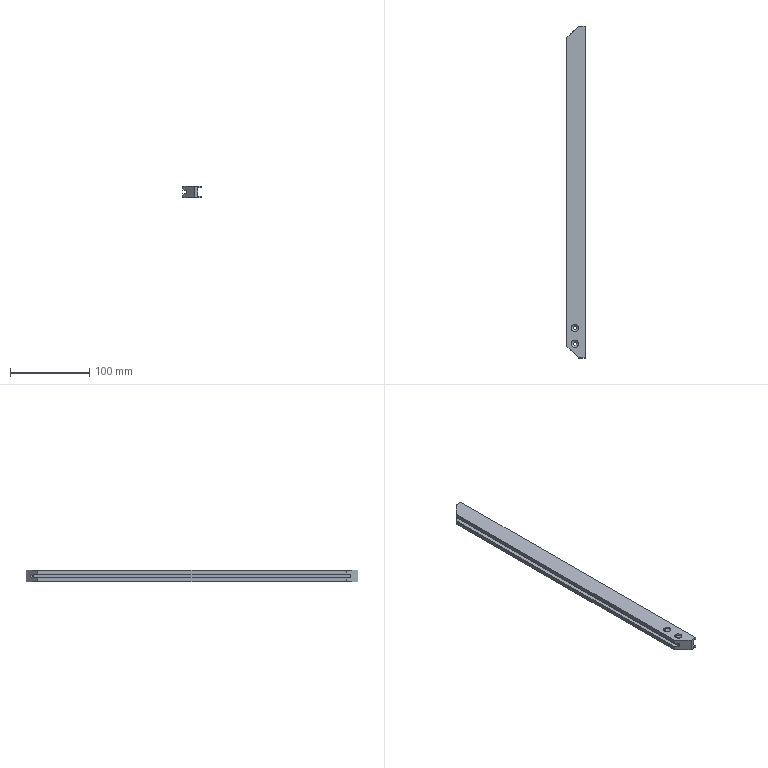Component | SolidWorks | AUTO-SpinDryWashing-01-03000005-1 | 1 solid | 34 faces | box 23 x 420 x 15 mm | volume 113031 mm3 | plane 16 | cylinder 12 | cone 6 | commonest cylinder face diameters 9.4 x4 4.5 x4 3.3 x2 2.5 x2 | material AISI 304
build123d program:
from build123d import *

# Parameters (mm, degrees)
BOSS_EXTRUDE1_DEPTH                                  = 210
CUT_EXTRUDE1_DEPTH                                   = 211.822
COUNTERSUNK_HOLE_FOR_M4_COUNTERSUNK_FLAT_D           = 4.5
COUNTERSUNK_HOLE_FOR_M4_COUNTERSUNK_FLAT_CSINK_D     = 9.4
COUNTERSUNK_HOLE_FOR_M4_COUNTERSUNK_FLAT_CSINK_ANGLE = 90
SKETCH7_W                                            = 15
SKETCH7_H                                            = 420
BOSS_EXTRUDE2_DEPTH                                  = 8
SKETCH8_W                                            = 10.5
SKETCH8_H                                            = 4
CUT_EXTRUDE2_DEPTH                                   = 421.469
M3_TAPPED_HOLE1_D                                    = 2.5
M3_TAPPED_HOLE1_DEPTH                                = 7.5
M3_TAPPED_HOLE1_TIP                                  = 0.7511
BOSS_EXTRUDE3_START                                  = 2
SKETCH12_R                                           = 2.25
BOSS_EXTRUDE3_DEPTH                                  = 2
SKETCH13_R                                           = 4.7
BOSS_EXTRUDE4_DEPTH                                  = 2
M4_TAPPED_HOLE1_D                                    = 3.3


with BuildPart() as part:
    # Sketch1 → Boss-Extrude1 (new, symmetric)
    with BuildSketch(Plane.XY):
        Polygon((0, 15), (0, 0), (11, 0), (11, 15), (8, 15), (8, 10), (3, 10), (3, 15), align=None)
    extrude(amount=BOSS_EXTRUDE1_DEPTH, both=True)

    # Sketch2 → Cut-Extrude1 (cut, through all)
    with BuildSketch(Plane.ZY):
        Polygon((-195, 15), (-210, 15), (-210, 0), align=None)
    cut_extrude1 = extrude(amount=-CUT_EXTRUDE1_DEPTH, mode=Mode.SUBTRACT)

    # Mirror1: Cut-Extrude1 across plane
    add(cut_extrude1.mirror(Plane.XY), mode=Mode.SUBTRACT)

    # Countersunk Hole for M4 Countersunk Flat (through all)
    with Locations(Plane.ZY):
        with Locations((-192, 5), (-172, 5)):
            CounterSinkHole(COUNTERSUNK_HOLE_FOR_M4_COUNTERSUNK_FLAT_D / 2, COUNTERSUNK_HOLE_FOR_M4_COUNTERSUNK_FLAT_CSINK_D / 2, counter_sink_angle=COUNTERSUNK_HOLE_FOR_M4_COUNTERSUNK_FLAT_CSINK_ANGLE)

    # Sketch7 → Boss-Extrude2 (add)
    with BuildSketch(Plane.XZ):
        with Locations((5.5, 0)):
            Rectangle(SKETCH7_W, SKETCH7_H)
    extrude(amount=BOSS_EXTRUDE2_DEPTH)

    # Sketch8 → Cut-Extrude2 (cut, through all)
    with BuildSketch(Plane.XY.offset(210)):
        with Locations((5.5, -6)):
            Rectangle(SKETCH8_W, SKETCH8_H)
    extrude(amount=-CUT_EXTRUDE2_DEPTH, mode=Mode.SUBTRACT)

    # M3 Tapped Hole1
    with Locations(Plane(origin=(0, -4, 0), x_dir=(-1, 0, 0), z_dir=(0, -1, 0))):
        with Locations((-5.5, -185)):
            Hole(M3_TAPPED_HOLE1_D / 2, depth=M3_TAPPED_HOLE1_DEPTH)
            with Locations((0, 0, -(M3_TAPPED_HOLE1_DEPTH + M3_TAPPED_HOLE1_TIP / 2))):  # 118° drill point
                Cone(0, M3_TAPPED_HOLE1_D / 2, M3_TAPPED_HOLE1_TIP, mode=Mode.SUBTRACT)

    # Sketch12 → Boss-Extrude3 (add)
    with BuildSketch(Plane(origin=(11, 0, 0), x_dir=(0, 0, -1), z_dir=(1, 0, 0)).offset(BOSS_EXTRUDE3_START)):
        Polygon((210, 0), (195, 15), (-195, 15), (-210, 0), align=None)
        with Locations(Location((172, 5, 0), (0, 0, 180))):
            Circle(SKETCH12_R, mode=Mode.SUBTRACT)
        with Locations(Location((192, 5, 0), (0, 0, 180))):
            Circle(SKETCH12_R, mode=Mode.SUBTRACT)
    extrude(amount=-BOSS_EXTRUDE3_DEPTH)

    # Sketch13 → Boss-Extrude4 (add)
    with BuildSketch(Plane.ZY):
        Polygon((210, 0), (195, 15), (-195, 15), (-210, 0), align=None)
        with Locations((-192, 5)):
            Circle(SKETCH13_R, mode=Mode.SUBTRACT)
        with Locations((-172, 5)):
            Circle(SKETCH13_R, mode=Mode.SUBTRACT)
    extrude(amount=BOSS_EXTRUDE4_DEPTH)

    # M4 Tapped Hole1 (through all)
    with Locations(Plane(origin=(0, 105, 105), x_dir=(1, 0, 0), z_dir=(0, 0.7071, 0.7071))):
        with Locations((5.5, -138.492)):
            Hole(M4_TAPPED_HOLE1_D / 2)


solid = part.part

# Placed as in the assembly
solid = solid.moved(Location((335, 588, 63), (-90, 0, 90)))
STEP:
#1=COLOUR_RGB('',0.7922,0.8196,0.9333);
#2=FILL_AREA_STYLE_COLOUR('',#1);
#3=FILL_AREA_STYLE('',(#2));
#4=SURFACE_STYLE_FILL_AREA(#3);
#5=SURFACE_SIDE_STYLE('',(#4));
#6=SURFACE_STYLE_USAGE(.BOTH.,#5);
#7=PRESENTATION_STYLE_ASSIGNMENT((#6));
#8=CARTESIAN_POINT('',(13.346,30.611,2.264));
#9=VERTEX_POINT('',#8);
#10=CARTESIAN_POINT('',(13.346,30.795,2.264));
#11=VERTEX_POINT('',#10);
#12=CARTESIAN_POINT('',(13.346,30.611,2.264));
#13=CARTESIAN_POINT('',(13.346,30.611,2.394));
#14=CARTESIAN_POINT('',(13.346,30.795,2.394));
#15=CARTESIAN_POINT('',(13.346,30.795,2.264));
#16=(BOUNDED_CURVE()B_SPLINE_CURVE(3,(#12,#13,#14,#15),.UNSPECIFIED.,.F.,.F.)B_SPLINE_CURVE_WITH_KNOTS((4,4),(3.142,6.283),.UNSPECIFIED.)CURVE()GEOMETRIC_REPRESENTATION_ITEM()RATIONAL_B_SPLINE_CURVE((1.,0.3333,0.3333,1.))REPRESENTATION_ITEM(''));
#17=EDGE_CURVE('',#9,#11,#16,.T.);
#18=ORIENTED_EDGE('',*,*,#17,.F.);
#19=CARTESIAN_POINT('',(12.865,31.093,2.264));
#20=VERTEX_POINT('',#19);
#21=CARTESIAN_POINT('',(12.865,31.093,2.264));
#22=DIRECTION('',(-0.7071,0.7071,-0.));
#23=VECTOR('',#22,39.37);
#24=LINE('',#21,#23);
#25=EDGE_CURVE('',#9,#20,#24,.T.);
#26=ORIENTED_EDGE('',*,*,#25,.T.);
#27=CARTESIAN_POINT('',(12.957,31.185,2.264));
#28=VERTEX_POINT('',#27);
#29=CARTESIAN_POINT('',(12.911,31.139,2.264));
#30=DIRECTION('',(-0.7071,0.7071,-0.));
#31=DIRECTION('',(0.7071,0.7071,0.));
#32=AXIS2_PLACEMENT_3D('',#29,#30,#31);
#33=CIRCLE('',#32,0.06496);
#34=EDGE_CURVE('',#20,#28,#33,.T.);
#35=ORIENTED_EDGE('',*,*,#34,.T.);
#36=CARTESIAN_POINT('',(12.957,31.185,2.264));
#37=DIRECTION('',(-0.7071,0.7071,-0.));
#38=VECTOR('',#37,39.37);
#39=LINE('',#36,#38);
#40=EDGE_CURVE('',#11,#28,#39,.T.);
#41=ORIENTED_EDGE('',*,*,#40,.F.);
#42=EDGE_LOOP('',(#18,#26,#35,#41));
#43=FACE_OUTER_BOUND('',#42,.T.);
#44=CARTESIAN_POINT('',(12.911,31.139,2.264));
#45=DIRECTION('',(-0.7071,0.7071,-0.));
#46=DIRECTION('',(0.7071,0.7071,0.));
#47=AXIS2_PLACEMENT_3D('',#44,#45,#46);
#48=CYLINDRICAL_SURFACE('',#47,0.06496);
#49=ADVANCED_FACE('',(#43),#48,.F.);
#50=CARTESIAN_POINT('',(12.992,16.193,2.559));
#51=VERTEX_POINT('',#50);
#52=CARTESIAN_POINT('',(12.992,16.563,2.559));
#53=VERTEX_POINT('',#52);
#54=CARTESIAN_POINT('',(12.992,16.378,2.559));
#55=DIRECTION('',(-0.,-0.,1.));
#56=DIRECTION('',(0.,1.,0.));
#57=AXIS2_PLACEMENT_3D('',#54,#55,#56);
#58=CIRCLE('',#57,0.185);
#59=EDGE_CURVE('',#51,#53,#58,.T.);
#60=ORIENTED_EDGE('',*,*,#59,.T.);
#61=CARTESIAN_POINT('',(12.992,16.563,2.48));
#62=VERTEX_POINT('',#61);
#63=CARTESIAN_POINT('',(12.992,16.563,2.559));
#64=DIRECTION('',(0.,0.,-1.));
#65=VECTOR('',#64,39.37);
#66=LINE('',#63,#65);
#67=EDGE_CURVE('',#53,#62,#66,.T.);
#68=ORIENTED_EDGE('',*,*,#67,.T.);
#69=CARTESIAN_POINT('',(12.992,16.193,2.48));
#70=VERTEX_POINT('',#69);
#71=CARTESIAN_POINT('',(12.992,16.378,2.48));
#72=DIRECTION('',(-0.,-0.,1.));
#73=DIRECTION('',(0.,1.,0.));
#74=AXIS2_PLACEMENT_3D('',#71,#72,#73);
#75=CIRCLE('',#74,0.185);
#76=EDGE_CURVE('',#70,#62,#75,.T.);
#77=ORIENTED_EDGE('',*,*,#76,.F.);
#78=CARTESIAN_POINT('',(12.992,16.193,2.559));
#79=DIRECTION('',(0.,0.,-1.));
#80=VECTOR('',#79,39.37);
#81=LINE('',#78,#80);
#82=EDGE_CURVE('',#51,#70,#81,.T.);
#83=ORIENTED_EDGE('',*,*,#82,.F.);
#84=EDGE_LOOP('',(#60,#68,#77,#83));
#85=FACE_OUTER_BOUND('',#84,.T.);
#86=CARTESIAN_POINT('',(12.992,16.378,2.559));
#87=DIRECTION('',(0.,0.,-1.));
#88=DIRECTION('',(0.,-1.,0.));
#89=AXIS2_PLACEMENT_3D('',#86,#87,#88);
#90=CYLINDRICAL_SURFACE('',#89,0.185);
#91=ADVANCED_FACE('',(#85),#90,.F.);
#92=CARTESIAN_POINT('',(12.992,15.406,2.559));
#93=VERTEX_POINT('',#92);
#94=CARTESIAN_POINT('',(12.992,15.776,2.559));
#95=VERTEX_POINT('',#94);
#96=CARTESIAN_POINT('',(12.992,15.591,2.559));
#97=DIRECTION('',(-0.,-0.,1.));
#98=DIRECTION('',(0.,1.,0.));
#99=AXIS2_PLACEMENT_3D('',#96,#97,#98);
#100=CIRCLE('',#99,0.185);
#101=EDGE_CURVE('',#93,#95,#100,.T.);
#102=ORIENTED_EDGE('',*,*,#101,.T.);
#103=CARTESIAN_POINT('',(12.992,15.776,2.48));
#104=VERTEX_POINT('',#103);
#105=CARTESIAN_POINT('',(12.992,15.776,2.559));
#106=DIRECTION('',(0.,0.,-1.));
#107=VECTOR('',#106,39.37);
#108=LINE('',#105,#107);
#109=EDGE_CURVE('',#95,#104,#108,.T.);
#110=ORIENTED_EDGE('',*,*,#109,.T.);
#111=CARTESIAN_POINT('',(12.992,15.406,2.48));
#112=VERTEX_POINT('',#111);
#113=CARTESIAN_POINT('',(12.992,15.591,2.48));
#114=DIRECTION('',(-0.,-0.,1.));
#115=DIRECTION('',(0.,1.,0.));
#116=AXIS2_PLACEMENT_3D('',#113,#114,#115);
#117=CIRCLE('',#116,0.185);
#118=EDGE_CURVE('',#112,#104,#117,.T.);
#119=ORIENTED_EDGE('',*,*,#118,.F.);
#120=CARTESIAN_POINT('',(12.992,15.406,2.559));
#121=DIRECTION('',(0.,0.,-1.));
#122=VECTOR('',#121,39.37);
#123=LINE('',#120,#122);
#124=EDGE_CURVE('',#93,#112,#123,.T.);
#125=ORIENTED_EDGE('',*,*,#124,.F.);
#126=EDGE_LOOP('',(#102,#110,#119,#125));
#127=FACE_OUTER_BOUND('',#126,.T.);
#128=CARTESIAN_POINT('',(12.992,15.591,2.559));
#129=DIRECTION('',(0.,0.,-1.));
#130=DIRECTION('',(0.,-1.,0.));
#131=AXIS2_PLACEMENT_3D('',#128,#129,#130);
#132=CYLINDRICAL_SURFACE('',#131,0.185);
#133=ADVANCED_FACE('',(#127),#132,.F.);
#134=CARTESIAN_POINT('',(13.051,30.482,2.264));
#135=VERTEX_POINT('',#134);
#136=CARTESIAN_POINT('',(13.051,30.384,2.264));
#137=VERTEX_POINT('',#136);
#138=CARTESIAN_POINT('',(13.051,30.433,2.264));
#139=DIRECTION('',(1.,0.,0.));
#140=DIRECTION('',(0.,-1.,0.));
#141=AXIS2_PLACEMENT_3D('',#138,#139,#140);
#142=CIRCLE('',#141,0.04921);
#143=EDGE_CURVE('',#135,#137,#142,.T.);
#144=ORIENTED_EDGE('',*,*,#143,.F.);
#145=CARTESIAN_POINT('',(13.346,30.482,2.264));
#146=VERTEX_POINT('',#145);
#147=CARTESIAN_POINT('',(13.346,30.482,2.264));
#148=DIRECTION('',(1.,0.,0.));
#149=VECTOR('',#148,39.37);
#150=LINE('',#147,#149);
#151=EDGE_CURVE('',#135,#146,#150,.T.);
#152=ORIENTED_EDGE('',*,*,#151,.T.);
#153=CARTESIAN_POINT('',(13.346,30.384,2.264));
#154=VERTEX_POINT('',#153);
#155=CARTESIAN_POINT('',(13.346,30.433,2.264));
#156=DIRECTION('',(1.,0.,0.));
#157=DIRECTION('',(0.,-1.,0.));
#158=AXIS2_PLACEMENT_3D('',#155,#156,#157);
#159=CIRCLE('',#158,0.04921);
#160=EDGE_CURVE('',#146,#154,#159,.T.);
#161=ORIENTED_EDGE('',*,*,#160,.T.);
#162=CARTESIAN_POINT('',(13.346,30.384,2.264));
#163=DIRECTION('',(1.,0.,0.));
#164=VECTOR('',#163,39.37);
#165=LINE('',#162,#164);
#166=EDGE_CURVE('',#137,#154,#165,.T.);
#167=ORIENTED_EDGE('',*,*,#166,.F.);
#168=EDGE_LOOP('',(#144,#152,#161,#167));
#169=FACE_OUTER_BOUND('',#168,.T.);
#170=CARTESIAN_POINT('',(13.346,30.433,2.264));
#171=DIRECTION('',(1.,0.,0.));
#172=DIRECTION('',(0.,-1.,0.));
#173=AXIS2_PLACEMENT_3D('',#170,#171,#172);
#174=CYLINDRICAL_SURFACE('',#173,0.04921);
#175=ADVANCED_FACE('',(#169),#174,.F.);
#176=CARTESIAN_POINT('',(13.022,30.433,2.264));
#177=VERTEX_POINT('',#176);
#178=CARTESIAN_POINT('',(13.051,30.384,2.264));
#179=DIRECTION('',(0.515,-0.8572,0.));
#180=VECTOR('',#179,39.37);
#181=LINE('',#178,#180);
#182=EDGE_CURVE('',#177,#137,#181,.T.);
#183=ORIENTED_EDGE('',*,*,#182,.F.);
#184=CARTESIAN_POINT('',(13.051,30.482,2.264));
#185=DIRECTION('',(0.515,0.8572,-0.));
#186=VECTOR('',#185,39.37);
#187=LINE('',#184,#186);
#188=EDGE_CURVE('',#177,#135,#187,.T.);
#189=ORIENTED_EDGE('',*,*,#188,.T.);
#190=ORIENTED_EDGE('',*,*,#143,.T.);
#191=EDGE_LOOP('',(#183,#189,#190));
#192=FACE_OUTER_BOUND('',#191,.T.);
#193=CARTESIAN_POINT('',(13.051,30.433,2.264));
#194=DIRECTION('',(1.,0.,0.));
#195=DIRECTION('',(0.,-1.,0.));
#196=AXIS2_PLACEMENT_3D('',#193,#194,#195);
#197=CONICAL_SURFACE('',#196,0.04921,1.03);
#198=ADVANCED_FACE('',(#192),#197,.F.);
#199=CARTESIAN_POINT('',(12.992,15.502,2.384));
#200=VERTEX_POINT('',#199);
#201=CARTESIAN_POINT('',(12.992,15.679,2.384));
#202=VERTEX_POINT('',#201);
#203=CARTESIAN_POINT('',(12.992,15.591,2.384));
#204=DIRECTION('',(-0.,-0.,1.));
#205=DIRECTION('',(0.,1.,0.));
#206=AXIS2_PLACEMENT_3D('',#203,#204,#205);
#207=CIRCLE('',#206,0.08858);
#208=EDGE_CURVE('',#200,#202,#207,.T.);
#209=ORIENTED_EDGE('',*,*,#208,.F.);
#210=CARTESIAN_POINT('',(12.992,15.406,2.48));
#211=DIRECTION('',(-0.,-0.7071,0.7071));
#212=VECTOR('',#211,39.37);
#213=LINE('',#210,#212);
#214=EDGE_CURVE('',#200,#112,#213,.T.);
#215=ORIENTED_EDGE('',*,*,#214,.T.);
#216=ORIENTED_EDGE('',*,*,#118,.T.);
#217=CARTESIAN_POINT('',(12.992,15.776,2.48));
#218=DIRECTION('',(-0.,0.7071,0.7071));
#219=VECTOR('',#218,39.37);
#220=LINE('',#217,#219);
#221=EDGE_CURVE('',#202,#104,#220,.T.);
#222=ORIENTED_EDGE('',*,*,#221,.F.);
#223=EDGE_LOOP('',(#209,#215,#216,#222));
#224=FACE_OUTER_BOUND('',#223,.T.);
#225=CARTESIAN_POINT('',(12.992,15.591,2.48));
#226=DIRECTION('',(-0.,-0.,1.));
#227=DIRECTION('',(0.,1.,0.));
#228=AXIS2_PLACEMENT_3D('',#225,#226,#227);
#229=CONICAL_SURFACE('',#228,0.185,0.7854);
#230=ADVANCED_FACE('',(#224),#229,.F.);
#231=CARTESIAN_POINT('',(12.992,15.679,1.969));
#232=VERTEX_POINT('',#231);
#233=CARTESIAN_POINT('',(12.992,15.502,1.969));
#234=VERTEX_POINT('',#233);
#235=CARTESIAN_POINT('',(12.992,15.591,1.969));
#236=DIRECTION('',(0.,0.,-1.));
#237=DIRECTION('',(0.,-1.,0.));
#238=AXIS2_PLACEMENT_3D('',#235,#236,#237);
#239=CIRCLE('',#238,0.08858);
#240=EDGE_CURVE('',#232,#234,#239,.T.);
#241=ORIENTED_EDGE('',*,*,#240,.T.);
#242=CARTESIAN_POINT('',(12.992,15.502,2.48));
#243=DIRECTION('',(-0.,-0.,1.));
#244=VECTOR('',#243,39.37);
#245=LINE('',#242,#244);
#246=EDGE_CURVE('',#234,#200,#245,.T.);
#247=ORIENTED_EDGE('',*,*,#246,.T.);
#248=ORIENTED_EDGE('',*,*,#208,.T.);
#249=CARTESIAN_POINT('',(12.992,15.679,2.48));
#250=DIRECTION('',(-0.,-0.,1.));
#251=VECTOR('',#250,39.37);
#252=LINE('',#249,#251);
#253=EDGE_CURVE('',#232,#202,#252,.T.);
#254=ORIENTED_EDGE('',*,*,#253,.F.);
#255=EDGE_LOOP('',(#241,#247,#248,#254));
#256=FACE_OUTER_BOUND('',#255,.T.);
#257=CARTESIAN_POINT('',(12.992,15.591,2.48));
#258=DIRECTION('',(-0.,-0.,1.));
#259=DIRECTION('',(0.,1.,0.));
#260=AXIS2_PLACEMENT_3D('',#257,#258,#259);
#261=CYLINDRICAL_SURFACE('',#260,0.08858);
#262=ADVANCED_FACE('',(#256),#261,.F.);
#263=CARTESIAN_POINT('',(12.992,16.289,2.384));
#264=VERTEX_POINT('',#263);
#265=CARTESIAN_POINT('',(12.992,16.467,2.384));
#266=VERTEX_POINT('',#265);
#267=CARTESIAN_POINT('',(12.992,16.378,2.384));
#268=DIRECTION('',(-0.,-0.,1.));
#269=DIRECTION('',(0.,1.,0.));
#270=AXIS2_PLACEMENT_3D('',#267,#268,#269);
#271=CIRCLE('',#270,0.08858);
#272=EDGE_CURVE('',#264,#266,#271,.T.);
#273=ORIENTED_EDGE('',*,*,#272,.F.);
#274=CARTESIAN_POINT('',(12.992,16.193,2.48));
#275=DIRECTION('',(-0.,-0.7071,0.7071));
#276=VECTOR('',#275,39.37);
#277=LINE('',#274,#276);
#278=EDGE_CURVE('',#264,#70,#277,.T.);
#279=ORIENTED_EDGE('',*,*,#278,.T.);
#280=ORIENTED_EDGE('',*,*,#76,.T.);
#281=CARTESIAN_POINT('',(12.992,16.563,2.48));
#282=DIRECTION('',(-0.,0.7071,0.7071));
#283=VECTOR('',#282,39.37);
#284=LINE('',#281,#283);
#285=EDGE_CURVE('',#266,#62,#284,.T.);
#286=ORIENTED_EDGE('',*,*,#285,.F.);
#287=EDGE_LOOP('',(#273,#279,#280,#286));
#288=FACE_OUTER_BOUND('',#287,.T.);
#289=CARTESIAN_POINT('',(12.992,16.378,2.48));
#290=DIRECTION('',(-0.,-0.,1.));
#291=DIRECTION('',(0.,1.,0.));
#292=AXIS2_PLACEMENT_3D('',#289,#290,#291);
#293=CONICAL_SURFACE('',#292,0.185,0.7854);
#294=ADVANCED_FACE('',(#288),#293,.F.);
#295=CARTESIAN_POINT('',(12.992,16.467,1.969));
#296=VERTEX_POINT('',#295);
#297=CARTESIAN_POINT('',(12.992,16.289,1.969));
#298=VERTEX_POINT('',#297);
#299=CARTESIAN_POINT('',(12.992,16.378,1.969));
#300=DIRECTION('',(0.,0.,-1.));
#301=DIRECTION('',(0.,-1.,0.));
#302=AXIS2_PLACEMENT_3D('',#299,#300,#301);
#303=CIRCLE('',#302,0.08858);
#304=EDGE_CURVE('',#296,#298,#303,.T.);
#305=ORIENTED_EDGE('',*,*,#304,.T.);
#306=CARTESIAN_POINT('',(12.992,16.289,2.48));
#307=DIRECTION('',(-0.,-0.,1.));
#308=VECTOR('',#307,39.37);
#309=LINE('',#306,#308);
#310=EDGE_CURVE('',#298,#264,#309,.T.);
#311=ORIENTED_EDGE('',*,*,#310,.T.);
#312=ORIENTED_EDGE('',*,*,#272,.T.);
#313=CARTESIAN_POINT('',(12.992,16.467,2.48));
#314=DIRECTION('',(-0.,-0.,1.));
#315=VECTOR('',#314,39.37);
#316=LINE('',#313,#315);
#317=EDGE_CURVE('',#296,#266,#316,.T.);
#318=ORIENTED_EDGE('',*,*,#317,.F.);
#319=EDGE_LOOP('',(#305,#311,#312,#318));
#320=FACE_OUTER_BOUND('',#319,.T.);
#321=CARTESIAN_POINT('',(12.992,16.378,2.48));
#322=DIRECTION('',(-0.,-0.,1.));
#323=DIRECTION('',(0.,1.,0.));
#324=AXIS2_PLACEMENT_3D('',#321,#322,#323);
#325=CYLINDRICAL_SURFACE('',#324,0.08858);
#326=ADVANCED_FACE('',(#320),#325,.F.);
#327=CARTESIAN_POINT('',(13.504,31.417,2.47));
#328=VERTEX_POINT('',#327);
#329=CARTESIAN_POINT('',(13.504,14.882,2.47));
#330=VERTEX_POINT('',#329);
#331=CARTESIAN_POINT('',(13.504,23.15,2.47));
#332=DIRECTION('',(0.,-1.,-0.));
#333=VECTOR('',#332,39.37);
#334=LINE('',#331,#333);
#335=EDGE_CURVE('',#328,#330,#334,.T.);
#336=ORIENTED_EDGE('',*,*,#335,.F.);
#337=CARTESIAN_POINT('',(13.504,31.417,2.559));
#338=VERTEX_POINT('',#337);
#339=CARTESIAN_POINT('',(13.504,31.417,2.559));
#340=DIRECTION('',(-0.,-0.,1.));
#341=VECTOR('',#340,39.37);
#342=LINE('',#339,#341);
#343=EDGE_CURVE('',#328,#338,#342,.T.);
#344=ORIENTED_EDGE('',*,*,#343,.T.);
#345=CARTESIAN_POINT('',(13.504,14.882,2.559));
#346=VERTEX_POINT('',#345);
#347=CARTESIAN_POINT('',(13.504,31.417,2.559));
#348=DIRECTION('',(0.,-1.,-0.));
#349=VECTOR('',#348,39.37);
#350=LINE('',#347,#349);
#351=EDGE_CURVE('',#338,#346,#350,.T.);
#352=ORIENTED_EDGE('',*,*,#351,.T.);
#353=CARTESIAN_POINT('',(13.504,14.882,2.559));
#354=DIRECTION('',(0.,0.,-1.));
#355=VECTOR('',#354,39.37);
#356=LINE('',#353,#355);
#357=EDGE_CURVE('',#346,#330,#356,.T.);
#358=ORIENTED_EDGE('',*,*,#357,.T.);
#359=EDGE_LOOP('',(#336,#344,#352,#358));
#360=FACE_OUTER_BOUND('',#359,.T.);
#361=CARTESIAN_POINT('',(13.504,23.15,2.48));
#362=DIRECTION('',(1.,0.,0.));
#363=DIRECTION('',(0.,-1.,-0.));
#364=AXIS2_PLACEMENT_3D('',#361,#362,#363);
#365=PLANE('',#364);
#366=ADVANCED_FACE('',(#360),#365,.T.);
#367=CARTESIAN_POINT('',(12.598,30.827,2.165));
#368=VERTEX_POINT('',#367);
#369=CARTESIAN_POINT('',(12.598,15.472,2.165));
#370=VERTEX_POINT('',#369);
#371=CARTESIAN_POINT('',(12.598,31.417,2.165));
#372=DIRECTION('',(0.,-1.,-0.));
#373=VECTOR('',#372,39.37);
#374=LINE('',#371,#373);
#375=EDGE_CURVE('',#368,#370,#374,.T.);
#376=ORIENTED_EDGE('',*,*,#375,.F.);
#377=CARTESIAN_POINT('',(12.598,30.827,1.969));
#378=VERTEX_POINT('',#377);
#379=CARTESIAN_POINT('',(12.598,30.827,2.047));
#380=DIRECTION('',(-0.,-0.,1.));
#381=VECTOR('',#380,39.37);
#382=LINE('',#379,#381);
#383=EDGE_CURVE('',#378,#368,#382,.T.);
#384=ORIENTED_EDGE('',*,*,#383,.F.);
#385=CARTESIAN_POINT('',(12.598,15.472,1.969));
#386=VERTEX_POINT('',#385);
#387=CARTESIAN_POINT('',(12.598,30.827,1.969));
#388=DIRECTION('',(-0.,1.,0.));
#389=VECTOR('',#388,39.37);
#390=LINE('',#387,#389);
#391=EDGE_CURVE('',#386,#378,#390,.T.);
#392=ORIENTED_EDGE('',*,*,#391,.F.);
#393=CARTESIAN_POINT('',(12.598,15.472,2.047));
#394=DIRECTION('',(-0.,-0.,1.));
#395=VECTOR('',#394,39.37);
#396=LINE('',#393,#395);
#397=EDGE_CURVE('',#386,#370,#396,.T.);
#398=ORIENTED_EDGE('',*,*,#397,.T.);
#399=EDGE_LOOP('',(#376,#384,#392,#398));
#400=FACE_OUTER_BOUND('',#399,.T.);
#401=CARTESIAN_POINT('',(12.598,31.417,2.48));
#402=DIRECTION('',(-1.,-0.,-0.));
#403=DIRECTION('',(-0.,1.,0.));
#404=AXIS2_PLACEMENT_3D('',#401,#402,#403);
#405=PLANE('',#404);
#406=ADVANCED_FACE('',(#400),#405,.T.);
#407=CARTESIAN_POINT('',(12.795,31.024,2.165));
#408=VERTEX_POINT('',#407);
#409=CARTESIAN_POINT('',(13.189,31.417,2.165));
#410=DIRECTION('',(0.7071,0.7071,-0.));
#411=VECTOR('',#410,39.37);
#412=LINE('',#409,#411);
#413=EDGE_CURVE('',#368,#408,#412,.T.);
#414=ORIENTED_EDGE('',*,*,#413,.F.);
#415=ORIENTED_EDGE('',*,*,#375,.T.);
#416=CARTESIAN_POINT('',(12.795,15.276,2.165));
#417=VERTEX_POINT('',#416);
#418=CARTESIAN_POINT('',(4.921,23.15,2.165));
#419=DIRECTION('',(0.7071,-0.7071,-0.));
#420=VECTOR('',#419,39.37);
#421=LINE('',#418,#420);
#422=EDGE_CURVE('',#370,#417,#421,.T.);
#423=ORIENTED_EDGE('',*,*,#422,.T.);
#424=CARTESIAN_POINT('',(12.795,31.417,2.165));
#425=DIRECTION('',(0.,-1.,-0.));
#426=VECTOR('',#425,39.37);
#427=LINE('',#424,#426);
#428=EDGE_CURVE('',#408,#417,#427,.T.);
#429=ORIENTED_EDGE('',*,*,#428,.F.);
#430=EDGE_LOOP('',(#414,#415,#423,#429));
#431=FACE_OUTER_BOUND('',#430,.T.);
#432=CARTESIAN_POINT('',(13.189,31.417,2.165));
#433=DIRECTION('',(-0.,0.,-1.));
#434=DIRECTION('',(-1.,-0.,0.));
#435=AXIS2_PLACEMENT_3D('',#432,#433,#434);
#436=PLANE('',#435);
#437=ADVANCED_FACE('',(#431),#436,.F.);
#438=CARTESIAN_POINT('',(12.795,31.024,2.362));
#439=VERTEX_POINT('',#438);
#440=CARTESIAN_POINT('',(12.795,15.276,2.362));
#441=VERTEX_POINT('',#440);
#442=CARTESIAN_POINT('',(12.795,31.417,2.362));
#443=DIRECTION('',(0.,-1.,-0.));
#444=VECTOR('',#443,39.37);
#445=LINE('',#442,#444);
#446=EDGE_CURVE('',#439,#441,#445,.T.);
#447=ORIENTED_EDGE('',*,*,#446,.F.);
#448=CARTESIAN_POINT('',(12.795,31.024,2.48));
#449=DIRECTION('',(0.,0.,-1.));
#450=VECTOR('',#449,39.37);
#451=LINE('',#448,#450);
#452=EDGE_CURVE('',#439,#408,#451,.T.);
#453=ORIENTED_EDGE('',*,*,#452,.T.);
#454=ORIENTED_EDGE('',*,*,#428,.T.);
#455=CARTESIAN_POINT('',(12.795,15.276,2.48));
#456=DIRECTION('',(0.,0.,-1.));
#457=VECTOR('',#456,39.37);
#458=LINE('',#455,#457);
#459=EDGE_CURVE('',#441,#417,#458,.T.);
#460=ORIENTED_EDGE('',*,*,#459,.F.);
#461=EDGE_LOOP('',(#447,#453,#454,#460));
#462=FACE_OUTER_BOUND('',#461,.T.);
#463=CARTESIAN_POINT('',(12.795,31.417,2.48));
#464=DIRECTION('',(-1.,-0.,-0.));
#465=DIRECTION('',(-0.,1.,0.));
#466=AXIS2_PLACEMENT_3D('',#463,#464,#465);
#467=PLANE('',#466);
#468=ADVANCED_FACE('',(#462),#467,.T.);
#469=CARTESIAN_POINT('',(12.598,30.827,2.362));
#470=VERTEX_POINT('',#469);
#471=CARTESIAN_POINT('',(12.598,15.472,2.362));
#472=VERTEX_POINT('',#471);
#473=CARTESIAN_POINT('',(12.598,31.417,2.362));
#474=DIRECTION('',(0.,-1.,-0.));
#475=VECTOR('',#474,39.37);
#476=LINE('',#473,#475);
#477=EDGE_CURVE('',#470,#472,#476,.T.);
#478=ORIENTED_EDGE('',*,*,#477,.F.);
#479=CARTESIAN_POINT('',(13.189,31.417,2.362));
#480=DIRECTION('',(0.7071,0.7071,0.));
#481=VECTOR('',#480,39.37);
#482=LINE('',#479,#481);
#483=EDGE_CURVE('',#470,#439,#482,.T.);
#484=ORIENTED_EDGE('',*,*,#483,.T.);
#485=ORIENTED_EDGE('',*,*,#446,.T.);
#486=CARTESIAN_POINT('',(4.921,23.15,2.362));
#487=DIRECTION('',(0.7071,-0.7071,0.));
#488=VECTOR('',#487,39.37);
#489=LINE('',#486,#488);
#490=EDGE_CURVE('',#472,#441,#489,.T.);
#491=ORIENTED_EDGE('',*,*,#490,.F.);
#492=EDGE_LOOP('',(#478,#484,#485,#491));
#493=FACE_OUTER_BOUND('',#492,.T.);
#494=CARTESIAN_POINT('',(13.189,31.417,2.362));
#495=DIRECTION('',(0.,0.,-1.));
#496=DIRECTION('',(-1.,-0.,-0.));
#497=AXIS2_PLACEMENT_3D('',#494,#495,#496);
#498=PLANE('',#497);
#499=ADVANCED_FACE('',(#493),#498,.T.);
#500=CARTESIAN_POINT('',(12.598,15.472,2.559));
#501=VERTEX_POINT('',#500);
#502=CARTESIAN_POINT('',(12.598,15.472,2.047));
#503=DIRECTION('',(-0.,-0.,1.));
#504=VECTOR('',#503,39.37);
#505=LINE('',#502,#504);
#506=EDGE_CURVE('',#472,#501,#505,.T.);
#507=ORIENTED_EDGE('',*,*,#506,.T.);
#508=CARTESIAN_POINT('',(12.598,30.827,2.559));
#509=VERTEX_POINT('',#508);
#510=CARTESIAN_POINT('',(12.598,30.827,2.559));
#511=DIRECTION('',(0.,-1.,-0.));
#512=VECTOR('',#511,39.37);
#513=LINE('',#510,#512);
#514=EDGE_CURVE('',#509,#501,#513,.T.);
#515=ORIENTED_EDGE('',*,*,#514,.F.);
#516=CARTESIAN_POINT('',(12.598,30.827,2.047));
#517=DIRECTION('',(-0.,-0.,1.));
#518=VECTOR('',#517,39.37);
#519=LINE('',#516,#518);
#520=EDGE_CURVE('',#470,#509,#519,.T.);
#521=ORIENTED_EDGE('',*,*,#520,.F.);
#522=ORIENTED_EDGE('',*,*,#477,.T.);
#523=EDGE_LOOP('',(#507,#515,#521,#522));
#524=FACE_OUTER_BOUND('',#523,.T.);
#525=CARTESIAN_POINT('',(12.598,31.417,2.48));
#526=DIRECTION('',(-1.,-0.,-0.));
#527=DIRECTION('',(-0.,1.,0.));
#528=AXIS2_PLACEMENT_3D('',#525,#526,#527);
#529=PLANE('',#528);
#530=ADVANCED_FACE('',(#524),#529,.T.);
#531=ORIENTED_EDGE('',*,*,#397,.F.);
#532=CARTESIAN_POINT('',(13.189,14.882,1.969));
#533=VERTEX_POINT('',#532);
#534=CARTESIAN_POINT('',(13.189,14.882,1.969));
#535=DIRECTION('',(-0.7071,0.7071,-0.));
#536=VECTOR('',#535,39.37);
#537=LINE('',#534,#536);
#538=EDGE_CURVE('',#533,#386,#537,.T.);
#539=ORIENTED_EDGE('',*,*,#538,.F.);
#540=CARTESIAN_POINT('',(13.189,14.882,2.559));
#541=VERTEX_POINT('',#540);
#542=CARTESIAN_POINT('',(13.189,14.882,2.48));
#543=DIRECTION('',(0.,0.,-1.));
#544=VECTOR('',#543,39.37);
#545=LINE('',#542,#544);
#546=EDGE_CURVE('',#541,#533,#545,.T.);
#547=ORIENTED_EDGE('',*,*,#546,.F.);
#548=CARTESIAN_POINT('',(13.189,14.882,2.559));
#549=DIRECTION('',(0.7071,-0.7071,0.));
#550=VECTOR('',#549,39.37);
#551=LINE('',#548,#550);
#552=EDGE_CURVE('',#501,#541,#551,.T.);
#553=ORIENTED_EDGE('',*,*,#552,.F.);
#554=ORIENTED_EDGE('',*,*,#506,.F.);
#555=ORIENTED_EDGE('',*,*,#490,.T.);
#556=ORIENTED_EDGE('',*,*,#459,.T.);
#557=ORIENTED_EDGE('',*,*,#422,.F.);
#558=EDGE_LOOP('',(#531,#539,#547,#553,#554,#555,#556,#557));
#559=FACE_OUTER_BOUND('',#558,.T.);
#560=CARTESIAN_POINT('',(13.189,14.882,2.047));
#561=DIRECTION('',(0.7071,0.7071,0.));
#562=DIRECTION('',(0.7071,-0.7071,0.));
#563=AXIS2_PLACEMENT_3D('',#560,#561,#562);
#564=PLANE('',#563);
#565=ADVANCED_FACE('',(#559),#564,.F.);
#566=CARTESIAN_POINT('',(12.911,31.139,2.264));
#567=DIRECTION('',(-0.7071,0.7071,-0.));
#568=DIRECTION('',(0.7071,0.7071,0.));
#569=AXIS2_PLACEMENT_3D('',#566,#567,#568);
#570=CIRCLE('',#569,0.06496);
#571=EDGE_CURVE('',#28,#20,#570,.T.);
#572=ORIENTED_EDGE('',*,*,#571,.F.);
#573=ORIENTED_EDGE('',*,*,#34,.F.);
#574=EDGE_LOOP('',(#572,#573));
#575=FACE_BOUND('',#574,.T.);
#576=ORIENTED_EDGE('',*,*,#413,.T.);
#577=ORIENTED_EDGE('',*,*,#452,.F.);
#578=ORIENTED_EDGE('',*,*,#483,.F.);
#579=ORIENTED_EDGE('',*,*,#520,.T.);
#580=CARTESIAN_POINT('',(13.189,31.417,2.559));
#581=VERTEX_POINT('',#580);
#582=CARTESIAN_POINT('',(13.189,31.417,2.559));
#583=DIRECTION('',(-0.7071,-0.7071,-0.));
#584=VECTOR('',#583,39.37);
#585=LINE('',#582,#584);
#586=EDGE_CURVE('',#581,#509,#585,.T.);
#587=ORIENTED_EDGE('',*,*,#586,.F.);
#588=CARTESIAN_POINT('',(13.189,31.417,1.969));
#589=VERTEX_POINT('',#588);
#590=CARTESIAN_POINT('',(13.189,31.417,2.48));
#591=DIRECTION('',(0.,0.,-1.));
#592=VECTOR('',#591,39.37);
#593=LINE('',#590,#592);
#594=EDGE_CURVE('',#581,#589,#593,.T.);
#595=ORIENTED_EDGE('',*,*,#594,.T.);
#596=CARTESIAN_POINT('',(13.189,31.417,1.969));
#597=DIRECTION('',(0.7071,0.7071,0.));
#598=VECTOR('',#597,39.37);
#599=LINE('',#596,#598);
#600=EDGE_CURVE('',#378,#589,#599,.T.);
#601=ORIENTED_EDGE('',*,*,#600,.F.);
#602=ORIENTED_EDGE('',*,*,#383,.T.);
#603=EDGE_LOOP('',(#576,#577,#578,#579,#587,#595,#601,#602));
#604=FACE_OUTER_BOUND('',#603,.T.);
#605=CARTESIAN_POINT('',(13.189,31.417,2.047));
#606=DIRECTION('',(-0.7071,0.7071,-0.));
#607=DIRECTION('',(0.7071,0.7071,0.));
#608=AXIS2_PLACEMENT_3D('',#605,#606,#607);
#609=PLANE('',#608);
#610=ADVANCED_FACE('',(#575,#604),#609,.T.);
#611=ORIENTED_EDGE('',*,*,#310,.F.);
#612=CARTESIAN_POINT('',(12.992,16.378,1.969));
#613=DIRECTION('',(0.,0.,-1.));
#614=DIRECTION('',(0.,-1.,0.));
#615=AXIS2_PLACEMENT_3D('',#612,#613,#614);
#616=CIRCLE('',#615,0.08858);
#617=EDGE_CURVE('',#298,#296,#616,.T.);
#618=ORIENTED_EDGE('',*,*,#617,.T.);
#619=ORIENTED_EDGE('',*,*,#317,.T.);
#620=CARTESIAN_POINT('',(12.992,16.378,2.384));
#621=DIRECTION('',(-0.,-0.,1.));
#622=DIRECTION('',(0.,1.,0.));
#623=AXIS2_PLACEMENT_3D('',#620,#621,#622);
#624=CIRCLE('',#623,0.08858);
#625=EDGE_CURVE('',#266,#264,#624,.T.);
#626=ORIENTED_EDGE('',*,*,#625,.T.);
#627=EDGE_LOOP('',(#611,#618,#619,#626));
#628=FACE_OUTER_BOUND('',#627,.T.);
#629=CARTESIAN_POINT('',(12.992,16.378,2.48));
#630=DIRECTION('',(-0.,-0.,1.));
#631=DIRECTION('',(0.,1.,0.));
#632=AXIS2_PLACEMENT_3D('',#629,#630,#631);
#633=CYLINDRICAL_SURFACE('',#632,0.08858);
#634=ADVANCED_FACE('',(#628),#633,.F.);
#635=ORIENTED_EDGE('',*,*,#278,.F.);
#636=ORIENTED_EDGE('',*,*,#625,.F.);
#637=ORIENTED_EDGE('',*,*,#285,.T.);
#638=CARTESIAN_POINT('',(12.992,16.378,2.48));
#639=DIRECTION('',(-0.,-0.,1.));
#640=DIRECTION('',(0.,1.,0.));
#641=AXIS2_PLACEMENT_3D('',#638,#639,#640);
#642=CIRCLE('',#641,0.185);
#643=EDGE_CURVE('',#62,#70,#642,.T.);
#644=ORIENTED_EDGE('',*,*,#643,.T.);
#645=EDGE_LOOP('',(#635,#636,#637,#644));
#646=FACE_OUTER_BOUND('',#645,.T.);
#647=CARTESIAN_POINT('',(12.992,16.378,2.48));
#648=DIRECTION('',(-0.,-0.,1.));
#649=DIRECTION('',(0.,1.,0.));
#650=AXIS2_PLACEMENT_3D('',#647,#648,#649);
#651=CONICAL_SURFACE('',#650,0.185,0.7854);
#652=ADVANCED_FACE('',(#646),#651,.F.);
#653=ORIENTED_EDGE('',*,*,#246,.F.);
#654=CARTESIAN_POINT('',(12.992,15.591,1.969));
#655=DIRECTION('',(0.,0.,-1.));
#656=DIRECTION('',(0.,-1.,0.));
#657=AXIS2_PLACEMENT_3D('',#654,#655,#656);
#658=CIRCLE('',#657,0.08858);
#659=EDGE_CURVE('',#234,#232,#658,.T.);
#660=ORIENTED_EDGE('',*,*,#659,.T.);
#661=ORIENTED_EDGE('',*,*,#253,.T.);
#662=CARTESIAN_POINT('',(12.992,15.591,2.384));
#663=DIRECTION('',(-0.,-0.,1.));
#664=DIRECTION('',(0.,1.,0.));
#665=AXIS2_PLACEMENT_3D('',#662,#663,#664);
#666=CIRCLE('',#665,0.08858);
#667=EDGE_CURVE('',#202,#200,#666,.T.);
#668=ORIENTED_EDGE('',*,*,#667,.T.);
#669=EDGE_LOOP('',(#653,#660,#661,#668));
#670=FACE_OUTER_BOUND('',#669,.T.);
#671=CARTESIAN_POINT('',(12.992,15.591,2.48));
#672=DIRECTION('',(-0.,-0.,1.));
#673=DIRECTION('',(0.,1.,0.));
#674=AXIS2_PLACEMENT_3D('',#671,#672,#673);
#675=CYLINDRICAL_SURFACE('',#674,0.08858);
#676=ADVANCED_FACE('',(#670),#675,.F.);
#677=ORIENTED_EDGE('',*,*,#214,.F.);
#678=ORIENTED_EDGE('',*,*,#667,.F.);
#679=ORIENTED_EDGE('',*,*,#221,.T.);
#680=CARTESIAN_POINT('',(12.992,15.591,2.48));
#681=DIRECTION('',(-0.,-0.,1.));
#682=DIRECTION('',(0.,1.,0.));
#683=AXIS2_PLACEMENT_3D('',#680,#681,#682);
#684=CIRCLE('',#683,0.185);
#685=EDGE_CURVE('',#104,#112,#684,.T.);
#686=ORIENTED_EDGE('',*,*,#685,.T.);
#687=EDGE_LOOP('',(#677,#678,#679,#686));
#688=FACE_OUTER_BOUND('',#687,.T.);
#689=CARTESIAN_POINT('',(12.992,15.591,2.48));
#690=DIRECTION('',(-0.,-0.,1.));
#691=DIRECTION('',(0.,1.,0.));
#692=AXIS2_PLACEMENT_3D('',#689,#690,#691);
#693=CONICAL_SURFACE('',#692,0.185,0.7854);
#694=ADVANCED_FACE('',(#688),#693,.F.);
#695=CARTESIAN_POINT('',(13.504,31.417,2.559));
#696=DIRECTION('',(-1.,-0.,-0.));
#697=VECTOR('',#696,39.37);
#698=LINE('',#695,#697);
#699=EDGE_CURVE('',#338,#581,#698,.T.);
#700=ORIENTED_EDGE('',*,*,#699,.T.);
#701=ORIENTED_EDGE('',*,*,#586,.T.);
#702=ORIENTED_EDGE('',*,*,#514,.T.);
#703=ORIENTED_EDGE('',*,*,#552,.T.);
#704=CARTESIAN_POINT('',(13.504,14.882,2.559));
#705=DIRECTION('',(-1.,-0.,-0.));
#706=VECTOR('',#705,39.37);
#707=LINE('',#704,#706);
#708=EDGE_CURVE('',#346,#541,#707,.T.);
#709=ORIENTED_EDGE('',*,*,#708,.F.);
#710=ORIENTED_EDGE('',*,*,#351,.F.);
#711=EDGE_LOOP('',(#700,#701,#702,#703,#709,#710));
#712=FACE_OUTER_BOUND('',#711,.T.);
#713=ORIENTED_EDGE('',*,*,#101,.F.);
#714=CARTESIAN_POINT('',(12.992,15.591,2.559));
#715=DIRECTION('',(-0.,-0.,1.));
#716=DIRECTION('',(0.,1.,0.));
#717=AXIS2_PLACEMENT_3D('',#714,#715,#716);
#718=CIRCLE('',#717,0.185);
#719=EDGE_CURVE('',#95,#93,#718,.T.);
#720=ORIENTED_EDGE('',*,*,#719,.F.);
#721=EDGE_LOOP('',(#713,#720));
#722=FACE_BOUND('',#721,.T.);
#723=ORIENTED_EDGE('',*,*,#59,.F.);
#724=CARTESIAN_POINT('',(12.992,16.378,2.559));
#725=DIRECTION('',(-0.,-0.,1.));
#726=DIRECTION('',(0.,1.,0.));
#727=AXIS2_PLACEMENT_3D('',#724,#725,#726);
#728=CIRCLE('',#727,0.185);
#729=EDGE_CURVE('',#53,#51,#728,.T.);
#730=ORIENTED_EDGE('',*,*,#729,.F.);
#731=EDGE_LOOP('',(#723,#730));
#732=FACE_BOUND('',#731,.T.);
#733=CARTESIAN_POINT('',(13.504,31.417,2.559));
#734=DIRECTION('',(0.,0.,-1.));
#735=DIRECTION('',(0.,-1.,-0.));
#736=AXIS2_PLACEMENT_3D('',#733,#734,#735);
#737=PLANE('',#736);
#738=ADVANCED_FACE('',(#712,#722,#732),#737,.F.);
#739=CARTESIAN_POINT('',(13.346,14.882,2.057));
#740=VERTEX_POINT('',#739);
#741=CARTESIAN_POINT('',(13.346,14.882,2.47));
#742=VERTEX_POINT('',#741);
#743=CARTESIAN_POINT('',(13.346,14.882,2.559));
#744=DIRECTION('',(-0.,-0.,1.));
#745=VECTOR('',#744,39.37);
#746=LINE('',#743,#745);
#747=EDGE_CURVE('',#740,#742,#746,.T.);
#748=ORIENTED_EDGE('',*,*,#747,.T.);
#749=CARTESIAN_POINT('',(13.504,14.882,2.47));
#750=DIRECTION('',(1.,0.,0.));
#751=VECTOR('',#750,39.37);
#752=LINE('',#749,#751);
#753=EDGE_CURVE('',#742,#330,#752,.T.);
#754=ORIENTED_EDGE('',*,*,#753,.T.);
#755=ORIENTED_EDGE('',*,*,#357,.F.);
#756=ORIENTED_EDGE('',*,*,#708,.T.);
#757=ORIENTED_EDGE('',*,*,#546,.T.);
#758=CARTESIAN_POINT('',(13.504,14.882,1.969));
#759=VERTEX_POINT('',#758);
#760=CARTESIAN_POINT('',(13.504,14.882,1.969));
#761=DIRECTION('',(-1.,-0.,-0.));
#762=VECTOR('',#761,39.37);
#763=LINE('',#760,#762);
#764=EDGE_CURVE('',#759,#533,#763,.T.);
#765=ORIENTED_EDGE('',*,*,#764,.F.);
#766=CARTESIAN_POINT('',(13.504,14.882,2.057));
#767=VERTEX_POINT('',#766);
#768=CARTESIAN_POINT('',(13.504,14.882,2.559));
#769=DIRECTION('',(0.,0.,-1.));
#770=VECTOR('',#769,39.37);
#771=LINE('',#768,#770);
#772=EDGE_CURVE('',#767,#759,#771,.T.);
#773=ORIENTED_EDGE('',*,*,#772,.F.);
#774=CARTESIAN_POINT('',(13.504,14.882,2.057));
#775=DIRECTION('',(-1.,-0.,-0.));
#776=VECTOR('',#775,39.37);
#777=LINE('',#774,#776);
#778=EDGE_CURVE('',#767,#740,#777,.T.);
#779=ORIENTED_EDGE('',*,*,#778,.T.);
#780=EDGE_LOOP('',(#748,#754,#755,#756,#757,#765,#773,#779));
#781=FACE_OUTER_BOUND('',#780,.T.);
#782=CARTESIAN_POINT('',(13.504,14.882,2.559));
#783=DIRECTION('',(-0.,1.,0.));
#784=DIRECTION('',(0.,0.,-1.));
#785=AXIS2_PLACEMENT_3D('',#782,#783,#784);
#786=PLANE('',#785);
#787=ADVANCED_FACE('',(#781),#786,.F.);
#788=ORIENTED_EDGE('',*,*,#764,.T.);
#789=ORIENTED_EDGE('',*,*,#538,.T.);
#790=ORIENTED_EDGE('',*,*,#391,.T.);
#791=ORIENTED_EDGE('',*,*,#600,.T.);
#792=CARTESIAN_POINT('',(13.504,31.417,1.969));
#793=VERTEX_POINT('',#792);
#794=CARTESIAN_POINT('',(13.504,31.417,1.969));
#795=DIRECTION('',(-1.,-0.,-0.));
#796=VECTOR('',#795,39.37);
#797=LINE('',#794,#796);
#798=EDGE_CURVE('',#793,#589,#797,.T.);
#799=ORIENTED_EDGE('',*,*,#798,.F.);
#800=CARTESIAN_POINT('',(13.504,31.417,1.969));
#801=DIRECTION('',(-0.,1.,0.));
#802=VECTOR('',#801,39.37);
#803=LINE('',#800,#802);
#804=EDGE_CURVE('',#759,#793,#803,.T.);
#805=ORIENTED_EDGE('',*,*,#804,.F.);
#806=EDGE_LOOP('',(#788,#789,#790,#791,#799,#805));
#807=FACE_OUTER_BOUND('',#806,.T.);
#808=ORIENTED_EDGE('',*,*,#304,.F.);
#809=ORIENTED_EDGE('',*,*,#617,.F.);
#810=EDGE_LOOP('',(#808,#809));
#811=FACE_BOUND('',#810,.T.);
#812=ORIENTED_EDGE('',*,*,#240,.F.);
#813=ORIENTED_EDGE('',*,*,#659,.F.);
#814=EDGE_LOOP('',(#812,#813));
#815=FACE_BOUND('',#814,.T.);
#816=CARTESIAN_POINT('',(13.504,31.417,1.969));
#817=DIRECTION('',(-0.,-0.,1.));
#818=DIRECTION('',(-0.,1.,0.));
#819=AXIS2_PLACEMENT_3D('',#816,#817,#818);
#820=PLANE('',#819);
#821=ADVANCED_FACE('',(#807,#811,#815),#820,.F.);
#822=ORIENTED_EDGE('',*,*,#343,.F.);
#823=CARTESIAN_POINT('',(13.346,31.417,2.47));
#824=VERTEX_POINT('',#823);
#825=CARTESIAN_POINT('',(13.504,31.417,2.47));
#826=DIRECTION('',(1.,0.,0.));
#827=VECTOR('',#826,39.37);
#828=LINE('',#825,#827);
#829=EDGE_CURVE('',#824,#328,#828,.T.);
#830=ORIENTED_EDGE('',*,*,#829,.F.);
#831=CARTESIAN_POINT('',(13.346,31.417,2.057));
#832=VERTEX_POINT('',#831);
#833=CARTESIAN_POINT('',(13.346,31.417,2.47));
#834=DIRECTION('',(-0.,-0.,1.));
#835=VECTOR('',#834,39.37);
#836=LINE('',#833,#835);
#837=EDGE_CURVE('',#832,#824,#836,.T.);
#838=ORIENTED_EDGE('',*,*,#837,.F.);
#839=CARTESIAN_POINT('',(13.504,31.417,2.057));
#840=VERTEX_POINT('',#839);
#841=CARTESIAN_POINT('',(13.504,31.417,2.057));
#842=DIRECTION('',(-1.,-0.,-0.));
#843=VECTOR('',#842,39.37);
#844=LINE('',#841,#843);
#845=EDGE_CURVE('',#840,#832,#844,.T.);
#846=ORIENTED_EDGE('',*,*,#845,.F.);
#847=CARTESIAN_POINT('',(13.504,31.417,2.559));
#848=DIRECTION('',(-0.,-0.,1.));
#849=VECTOR('',#848,39.37);
#850=LINE('',#847,#849);
#851=EDGE_CURVE('',#793,#840,#850,.T.);
#852=ORIENTED_EDGE('',*,*,#851,.F.);
#853=ORIENTED_EDGE('',*,*,#798,.T.);
#854=ORIENTED_EDGE('',*,*,#594,.F.);
#855=ORIENTED_EDGE('',*,*,#699,.F.);
#856=EDGE_LOOP('',(#822,#830,#838,#846,#852,#853,#854,#855));
#857=FACE_OUTER_BOUND('',#856,.T.);
#858=CARTESIAN_POINT('',(13.504,31.417,2.559));
#859=DIRECTION('',(0.,-1.,-0.));
#860=DIRECTION('',(-0.,-0.,1.));
#861=AXIS2_PLACEMENT_3D('',#858,#859,#860);
#862=PLANE('',#861);
#863=ADVANCED_FACE('',(#857),#862,.F.);
#864=CARTESIAN_POINT('',(13.504,23.15,2.057));
#865=DIRECTION('',(-0.,1.,0.));
#866=VECTOR('',#865,39.37);
#867=LINE('',#864,#866);
#868=EDGE_CURVE('',#767,#840,#867,.T.);
#869=ORIENTED_EDGE('',*,*,#868,.F.);
#870=ORIENTED_EDGE('',*,*,#772,.T.);
#871=ORIENTED_EDGE('',*,*,#804,.T.);
#872=ORIENTED_EDGE('',*,*,#851,.T.);
#873=EDGE_LOOP('',(#869,#870,#871,#872));
#874=FACE_OUTER_BOUND('',#873,.T.);
#875=CARTESIAN_POINT('',(13.504,23.15,2.48));
#876=DIRECTION('',(1.,0.,0.));
#877=DIRECTION('',(0.,-1.,-0.));
#878=AXIS2_PLACEMENT_3D('',#875,#876,#877);
#879=PLANE('',#878);
#880=ADVANCED_FACE('',(#874),#879,.T.);
#881=CARTESIAN_POINT('',(13.346,30.795,2.264));
#882=CARTESIAN_POINT('',(13.346,30.795,2.134));
#883=CARTESIAN_POINT('',(13.346,30.611,2.134));
#884=CARTESIAN_POINT('',(13.346,30.611,2.264));
#885=(BOUNDED_CURVE()B_SPLINE_CURVE(3,(#881,#882,#883,#884),.UNSPECIFIED.,.F.,.F.)B_SPLINE_CURVE_WITH_KNOTS((4,4),(0.,3.142),.UNSPECIFIED.)CURVE()GEOMETRIC_REPRESENTATION_ITEM()RATIONAL_B_SPLINE_CURVE((1.,0.3333,0.3333,1.))REPRESENTATION_ITEM(''));
#886=EDGE_CURVE('',#11,#9,#885,.T.);
#887=ORIENTED_EDGE('',*,*,#886,.T.);
#888=ORIENTED_EDGE('',*,*,#17,.T.);
#889=EDGE_LOOP('',(#887,#888));
#890=FACE_BOUND('',#889,.T.);
#891=CARTESIAN_POINT('',(13.346,30.433,2.264));
#892=DIRECTION('',(1.,0.,0.));
#893=DIRECTION('',(0.,-1.,0.));
#894=AXIS2_PLACEMENT_3D('',#891,#892,#893);
#895=CIRCLE('',#894,0.04921);
#896=EDGE_CURVE('',#154,#146,#895,.T.);
#897=ORIENTED_EDGE('',*,*,#896,.F.);
#898=ORIENTED_EDGE('',*,*,#160,.F.);
#899=EDGE_LOOP('',(#897,#898));
#900=FACE_BOUND('',#899,.T.);
#901=CARTESIAN_POINT('',(13.346,14.882,2.057));
#902=DIRECTION('',(-0.,1.,0.));
#903=VECTOR('',#902,39.37);
#904=LINE('',#901,#903);
#905=EDGE_CURVE('',#740,#832,#904,.T.);
#906=ORIENTED_EDGE('',*,*,#905,.T.);
#907=ORIENTED_EDGE('',*,*,#837,.T.);
#908=CARTESIAN_POINT('',(13.346,14.882,2.47));
#909=DIRECTION('',(-0.,1.,0.));
#910=VECTOR('',#909,39.37);
#911=LINE('',#908,#910);
#912=EDGE_CURVE('',#742,#824,#911,.T.);
#913=ORIENTED_EDGE('',*,*,#912,.F.);
#914=ORIENTED_EDGE('',*,*,#747,.F.);
#915=EDGE_LOOP('',(#906,#907,#913,#914));
#916=FACE_OUTER_BOUND('',#915,.T.);
#917=CARTESIAN_POINT('',(13.346,14.882,2.47));
#918=DIRECTION('',(-1.,-0.,-0.));
#919=DIRECTION('',(-0.,1.,0.));
#920=AXIS2_PLACEMENT_3D('',#917,#918,#919);
#921=PLANE('',#920);
#922=ADVANCED_FACE('',(#890,#900,#916),#921,.F.);
#923=ORIENTED_EDGE('',*,*,#912,.T.);
#924=ORIENTED_EDGE('',*,*,#829,.T.);
#925=ORIENTED_EDGE('',*,*,#335,.T.);
#926=ORIENTED_EDGE('',*,*,#753,.F.);
#927=EDGE_LOOP('',(#923,#924,#925,#926));
#928=FACE_OUTER_BOUND('',#927,.T.);
#929=CARTESIAN_POINT('',(13.504,14.882,2.47));
#930=DIRECTION('',(-0.,-0.,1.));
#931=DIRECTION('',(1.,0.,0.));
#932=AXIS2_PLACEMENT_3D('',#929,#930,#931);
#933=PLANE('',#932);
#934=ADVANCED_FACE('',(#928),#933,.F.);
#935=ORIENTED_EDGE('',*,*,#868,.T.);
#936=ORIENTED_EDGE('',*,*,#845,.T.);
#937=ORIENTED_EDGE('',*,*,#905,.F.);
#938=ORIENTED_EDGE('',*,*,#778,.F.);
#939=EDGE_LOOP('',(#935,#936,#937,#938));
#940=FACE_OUTER_BOUND('',#939,.T.);
#941=CARTESIAN_POINT('',(13.504,14.882,2.057));
#942=DIRECTION('',(0.,0.,-1.));
#943=DIRECTION('',(0.,-1.,-0.));
#944=AXIS2_PLACEMENT_3D('',#941,#942,#943);
#945=PLANE('',#944);
#946=ADVANCED_FACE('',(#940),#945,.F.);
#947=ORIENTED_EDGE('',*,*,#188,.F.);
#948=ORIENTED_EDGE('',*,*,#182,.T.);
#949=CARTESIAN_POINT('',(13.051,30.433,2.264));
#950=DIRECTION('',(1.,0.,0.));
#951=DIRECTION('',(0.,-1.,0.));
#952=AXIS2_PLACEMENT_3D('',#949,#950,#951);
#953=CIRCLE('',#952,0.04921);
#954=EDGE_CURVE('',#137,#135,#953,.T.);
#955=ORIENTED_EDGE('',*,*,#954,.T.);
#956=EDGE_LOOP('',(#947,#948,#955));
#957=FACE_OUTER_BOUND('',#956,.T.);
#958=CARTESIAN_POINT('',(13.051,30.433,2.264));
#959=DIRECTION('',(1.,0.,0.));
#960=DIRECTION('',(0.,-1.,0.));
#961=AXIS2_PLACEMENT_3D('',#958,#959,#960);
#962=CONICAL_SURFACE('',#961,0.04921,1.03);
#963=ADVANCED_FACE('',(#957),#962,.F.);
#964=ORIENTED_EDGE('',*,*,#151,.F.);
#965=ORIENTED_EDGE('',*,*,#954,.F.);
#966=ORIENTED_EDGE('',*,*,#166,.T.);
#967=ORIENTED_EDGE('',*,*,#896,.T.);
#968=EDGE_LOOP('',(#964,#965,#966,#967));
#969=FACE_OUTER_BOUND('',#968,.T.);
#970=CARTESIAN_POINT('',(13.346,30.433,2.264));
#971=DIRECTION('',(1.,0.,0.));
#972=DIRECTION('',(0.,-1.,0.));
#973=AXIS2_PLACEMENT_3D('',#970,#971,#972);
#974=CYLINDRICAL_SURFACE('',#973,0.04921);
#975=ADVANCED_FACE('',(#969),#974,.F.);
#976=ORIENTED_EDGE('',*,*,#109,.F.);
#977=ORIENTED_EDGE('',*,*,#719,.T.);
#978=ORIENTED_EDGE('',*,*,#124,.T.);
#979=ORIENTED_EDGE('',*,*,#685,.F.);
#980=EDGE_LOOP('',(#976,#977,#978,#979));
#981=FACE_OUTER_BOUND('',#980,.T.);
#982=CARTESIAN_POINT('',(12.992,15.591,2.559));
#983=DIRECTION('',(0.,0.,-1.));
#984=DIRECTION('',(0.,-1.,0.));
#985=AXIS2_PLACEMENT_3D('',#982,#983,#984);
#986=CYLINDRICAL_SURFACE('',#985,0.185);
#987=ADVANCED_FACE('',(#981),#986,.F.);
#988=ORIENTED_EDGE('',*,*,#67,.F.);
#989=ORIENTED_EDGE('',*,*,#729,.T.);
#990=ORIENTED_EDGE('',*,*,#82,.T.);
#991=ORIENTED_EDGE('',*,*,#643,.F.);
#992=EDGE_LOOP('',(#988,#989,#990,#991));
#993=FACE_OUTER_BOUND('',#992,.T.);
#994=CARTESIAN_POINT('',(12.992,16.378,2.559));
#995=DIRECTION('',(0.,0.,-1.));
#996=DIRECTION('',(0.,-1.,0.));
#997=AXIS2_PLACEMENT_3D('',#994,#995,#996);
#998=CYLINDRICAL_SURFACE('',#997,0.185);
#999=ADVANCED_FACE('',(#993),#998,.F.);
#1000=ORIENTED_EDGE('',*,*,#25,.F.);
#1001=ORIENTED_EDGE('',*,*,#886,.F.);
#1002=ORIENTED_EDGE('',*,*,#40,.T.);
#1003=ORIENTED_EDGE('',*,*,#571,.T.);
#1004=EDGE_LOOP('',(#1000,#1001,#1002,#1003));
#1005=FACE_OUTER_BOUND('',#1004,.T.);
#1006=CARTESIAN_POINT('',(12.911,31.139,2.264));
#1007=DIRECTION('',(-0.7071,0.7071,-0.));
#1008=DIRECTION('',(0.7071,0.7071,0.));
#1009=AXIS2_PLACEMENT_3D('',#1006,#1007,#1008);
#1010=CYLINDRICAL_SURFACE('',#1009,0.06496);
#1011=ADVANCED_FACE('',(#1005),#1010,.F.);
#1012=CLOSED_SHELL('',(#49,#91,#133,#175,#198,#230,#262,#294,#326,#366,#406,#437,#468,#499,#530,#565,#610,#634,#652,#676,#694,#738,#787,#821,#863,#880,#922,#934,#946,#963,#975,#987,#999,#1011));
#1013=MANIFOLD_SOLID_BREP('',#1012);
#1014=STYLED_ITEM('',(#7),#1013);
#1015=(LENGTH_UNIT()NAMED_UNIT(*)SI_UNIT($,.METRE.));
#1016=LENGTH_MEASURE_WITH_UNIT(LENGTH_MEASURE(0.0254),#1015);
#1017=DIMENSIONAL_EXPONENTS(1.,0.,0.,0.,0.,0.,0.);
#1018=(CONVERSION_BASED_UNIT('',#1016)LENGTH_UNIT()NAMED_UNIT(#1017));
#1019=UNCERTAINTY_MEASURE_WITH_UNIT(LENGTH_MEASURE(0.00001),#1018,'','');
#1020=(NAMED_UNIT(*)PLANE_ANGLE_UNIT()SI_UNIT($,.RADIAN.));
#1021=(NAMED_UNIT(*)SI_UNIT($,.STERADIAN.)SOLID_ANGLE_UNIT());
#1022=(GEOMETRIC_REPRESENTATION_CONTEXT(3)GLOBAL_UNCERTAINTY_ASSIGNED_CONTEXT((#1019))GLOBAL_UNIT_ASSIGNED_CONTEXT((#1018,#1020,#1021))REPRESENTATION_CONTEXT('',''));
#1023=MECHANICAL_DESIGN_GEOMETRIC_PRESENTATION_REPRESENTATION('',(#1014),#1022);
#1024=CARTESIAN_POINT('',(0.,0.,0.));
#1025=DIRECTION('',(0.,0.,1.));
#1026=DIRECTION('',(1.,0.,0.));
#1027=AXIS2_PLACEMENT_3D('',#1024,#1025,#1026);
#1028=(LENGTH_UNIT()NAMED_UNIT(*)SI_UNIT($,.METRE.));
#1029=LENGTH_MEASURE_WITH_UNIT(LENGTH_MEASURE(0.0254),#1028);
#1030=DIMENSIONAL_EXPONENTS(1.,0.,0.,0.,0.,0.,0.);
#1031=(CONVERSION_BASED_UNIT('',#1029)LENGTH_UNIT()NAMED_UNIT(#1030));
#1032=UNCERTAINTY_MEASURE_WITH_UNIT(LENGTH_MEASURE(0.00001),#1031,'','');
#1033=(NAMED_UNIT(*)PLANE_ANGLE_UNIT()SI_UNIT($,.RADIAN.));
#1034=(NAMED_UNIT(*)SI_UNIT($,.STERADIAN.)SOLID_ANGLE_UNIT());
#1035=(GEOMETRIC_REPRESENTATION_CONTEXT(3)GLOBAL_UNCERTAINTY_ASSIGNED_CONTEXT((#1032))GLOBAL_UNIT_ASSIGNED_CONTEXT((#1031,#1033,#1034))REPRESENTATION_CONTEXT('',''));
#1036=ADVANCED_BREP_SHAPE_REPRESENTATION('',(#1013,#1027),#1035);
#1037=PRESENTATION_LAYER_ASSIGNMENT('','',(#1014));